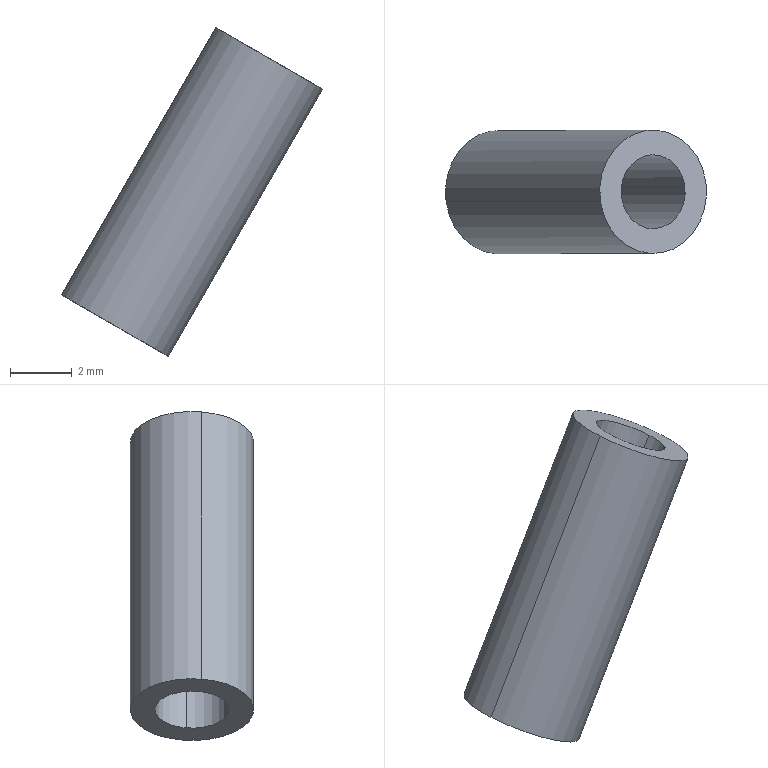Component | SolidWorks | WaterPipe5-1 | 1 solid | 6 faces | box 8.46 x 4 x 10.66 mm | volume 80 mm3 | cylinder 4 | plane 2 | commonest cylinder face diameters 2.4 x2 4 x2
build123d program:
from build123d import *

# Parameters (mm, degrees)
SCAN_THIN_FEATURE1_PROFILE_R   = 2
SCAN_THIN_FEATURE1_PROFILE_R_2 = 1.2


with BuildPart() as part:
    # Scan-Thin Feature1: sweep along a path in Sketch1
    with BuildLine(Plane.XY) as scan_thin_feature1_path:
        Line((0, 0), (10, 0))
    # Scan-Thin Feature1 profile (on start of the path) → Scan-Thin Feature1 (sweep)
    with BuildSketch(Plane(origin=(0, 0, 0), x_dir=(0, 0, 1), z_dir=(1, 0, 0))):
        Circle(SCAN_THIN_FEATURE1_PROFILE_R)
        Circle(SCAN_THIN_FEATURE1_PROFILE_R_2, mode=Mode.SUBTRACT)
    sweep(path=scan_thin_feature1_path.line)


solid = part.part

# Placed as in the assembly
solid = solid.moved(Location((35.951, 33.561, 104.495), (-176.489, 59.953, -3.04)))
STEP:
#1=CARTESIAN_POINT('',(1.375,1.314,4.137));
#2=VERTEX_POINT('',#1);
#3=CARTESIAN_POINT('',(1.456,1.329,4.091));
#4=VERTEX_POINT('',#3);
#5=CARTESIAN_POINT('',(1.415,1.321,4.114));
#6=DIRECTION('',(0.5,0.,0.866));
#7=DIRECTION('',(0.8553,0.1566,-0.4938));
#8=AXIS2_PLACEMENT_3D('',#5,#6,#7);
#9=CIRCLE('',#8,0.04724);
#10=EDGE_CURVE('',#2,#4,#9,.T.);
#11=ORIENTED_EDGE('',*,*,#10,.F.);
#12=CARTESIAN_POINT('',(1.572,1.314,4.478));
#13=VERTEX_POINT('',#12);
#14=CARTESIAN_POINT('',(1.375,1.314,4.137));
#15=DIRECTION('',(0.5,0.,0.866));
#16=VECTOR('',#15,39.37);
#17=LINE('',#14,#16);
#18=EDGE_CURVE('',#2,#13,#17,.T.);
#19=ORIENTED_EDGE('',*,*,#18,.T.);
#20=CARTESIAN_POINT('',(1.653,1.329,4.432));
#21=VERTEX_POINT('',#20);
#22=CARTESIAN_POINT('',(1.612,1.321,4.455));
#23=DIRECTION('',(0.5,0.,0.866));
#24=DIRECTION('',(0.8553,0.1566,-0.4938));
#25=AXIS2_PLACEMENT_3D('',#22,#23,#24);
#26=CIRCLE('',#25,0.04724);
#27=EDGE_CURVE('',#13,#21,#26,.T.);
#28=ORIENTED_EDGE('',*,*,#27,.T.);
#29=CARTESIAN_POINT('',(1.456,1.329,4.091));
#30=DIRECTION('',(0.5,0.,0.866));
#31=VECTOR('',#30,39.37);
#32=LINE('',#29,#31);
#33=EDGE_CURVE('',#4,#21,#32,.T.);
#34=ORIENTED_EDGE('',*,*,#33,.F.);
#35=EDGE_LOOP('',(#11,#19,#28,#34));
#36=FACE_OUTER_BOUND('',#35,.T.);
#37=CARTESIAN_POINT('',(1.415,1.321,4.114));
#38=DIRECTION('',(0.5,0.,0.866));
#39=DIRECTION('',(0.8553,0.1566,-0.4938));
#40=AXIS2_PLACEMENT_3D('',#37,#38,#39);
#41=CYLINDRICAL_SURFACE('',#40,0.04724);
#42=ADVANCED_FACE('',(#36),#41,.F.);
#43=CARTESIAN_POINT('',(1.483,1.334,4.075));
#44=VERTEX_POINT('',#43);
#45=CARTESIAN_POINT('',(1.348,1.309,4.153));
#46=VERTEX_POINT('',#45);
#47=CARTESIAN_POINT('',(1.415,1.321,4.114));
#48=DIRECTION('',(0.5,0.,0.866));
#49=DIRECTION('',(0.8553,0.1566,-0.4938));
#50=AXIS2_PLACEMENT_3D('',#47,#48,#49);
#51=CIRCLE('',#50,0.07874);
#52=EDGE_CURVE('',#44,#46,#51,.T.);
#53=ORIENTED_EDGE('',*,*,#52,.T.);
#54=CARTESIAN_POINT('',(1.545,1.309,4.494));
#55=VERTEX_POINT('',#54);
#56=CARTESIAN_POINT('',(1.348,1.309,4.153));
#57=DIRECTION('',(0.5,0.,0.866));
#58=VECTOR('',#57,39.37);
#59=LINE('',#56,#58);
#60=EDGE_CURVE('',#46,#55,#59,.T.);
#61=ORIENTED_EDGE('',*,*,#60,.T.);
#62=CARTESIAN_POINT('',(1.68,1.334,4.416));
#63=VERTEX_POINT('',#62);
#64=CARTESIAN_POINT('',(1.612,1.321,4.455));
#65=DIRECTION('',(0.5,0.,0.866));
#66=DIRECTION('',(0.8553,0.1566,-0.4938));
#67=AXIS2_PLACEMENT_3D('',#64,#65,#66);
#68=CIRCLE('',#67,0.07874);
#69=EDGE_CURVE('',#63,#55,#68,.T.);
#70=ORIENTED_EDGE('',*,*,#69,.F.);
#71=CARTESIAN_POINT('',(1.483,1.334,4.075));
#72=DIRECTION('',(0.5,0.,0.866));
#73=VECTOR('',#72,39.37);
#74=LINE('',#71,#73);
#75=EDGE_CURVE('',#44,#63,#74,.T.);
#76=ORIENTED_EDGE('',*,*,#75,.F.);
#77=EDGE_LOOP('',(#53,#61,#70,#76));
#78=FACE_OUTER_BOUND('',#77,.T.);
#79=CARTESIAN_POINT('',(1.415,1.321,4.114));
#80=DIRECTION('',(0.5,0.,0.866));
#81=DIRECTION('',(0.8553,0.1566,-0.4938));
#82=AXIS2_PLACEMENT_3D('',#79,#80,#81);
#83=CYLINDRICAL_SURFACE('',#82,0.07874);
#84=ADVANCED_FACE('',(#78),#83,.T.);
#85=ORIENTED_EDGE('',*,*,#60,.F.);
#86=CARTESIAN_POINT('',(1.415,1.321,4.114));
#87=DIRECTION('',(0.5,0.,0.866));
#88=DIRECTION('',(0.8553,0.1566,-0.4938));
#89=AXIS2_PLACEMENT_3D('',#86,#87,#88);
#90=CIRCLE('',#89,0.07874);
#91=EDGE_CURVE('',#46,#44,#90,.T.);
#92=ORIENTED_EDGE('',*,*,#91,.T.);
#93=ORIENTED_EDGE('',*,*,#75,.T.);
#94=CARTESIAN_POINT('',(1.612,1.321,4.455));
#95=DIRECTION('',(0.5,0.,0.866));
#96=DIRECTION('',(0.8553,0.1566,-0.4938));
#97=AXIS2_PLACEMENT_3D('',#94,#95,#96);
#98=CIRCLE('',#97,0.07874);
#99=EDGE_CURVE('',#55,#63,#98,.T.);
#100=ORIENTED_EDGE('',*,*,#99,.F.);
#101=EDGE_LOOP('',(#85,#92,#93,#100));
#102=FACE_OUTER_BOUND('',#101,.T.);
#103=CARTESIAN_POINT('',(1.415,1.321,4.114));
#104=DIRECTION('',(0.5,0.,0.866));
#105=DIRECTION('',(0.8553,0.1566,-0.4938));
#106=AXIS2_PLACEMENT_3D('',#103,#104,#105);
#107=CYLINDRICAL_SURFACE('',#106,0.07874);
#108=ADVANCED_FACE('',(#102),#107,.T.);
#109=CARTESIAN_POINT('',(1.612,1.321,4.455));
#110=DIRECTION('',(0.5,0.,0.866));
#111=DIRECTION('',(0.8553,0.1566,-0.4938));
#112=AXIS2_PLACEMENT_3D('',#109,#110,#111);
#113=CIRCLE('',#112,0.04724);
#114=EDGE_CURVE('',#21,#13,#113,.T.);
#115=ORIENTED_EDGE('',*,*,#114,.F.);
#116=ORIENTED_EDGE('',*,*,#27,.F.);
#117=EDGE_LOOP('',(#115,#116));
#118=FACE_BOUND('',#117,.T.);
#119=ORIENTED_EDGE('',*,*,#69,.T.);
#120=ORIENTED_EDGE('',*,*,#99,.T.);
#121=EDGE_LOOP('',(#119,#120));
#122=FACE_OUTER_BOUND('',#121,.T.);
#123=CARTESIAN_POINT('',(1.612,1.321,4.455));
#124=DIRECTION('',(0.5,0.,0.866));
#125=DIRECTION('',(0.8553,0.1566,-0.4938));
#126=AXIS2_PLACEMENT_3D('',#123,#124,#125);
#127=PLANE('',#126);
#128=ADVANCED_FACE('',(#118,#122),#127,.T.);
#129=CARTESIAN_POINT('',(1.415,1.321,4.114));
#130=DIRECTION('',(0.5,0.,0.866));
#131=DIRECTION('',(0.8553,0.1566,-0.4938));
#132=AXIS2_PLACEMENT_3D('',#129,#130,#131);
#133=CIRCLE('',#132,0.04724);
#134=EDGE_CURVE('',#4,#2,#133,.T.);
#135=ORIENTED_EDGE('',*,*,#134,.T.);
#136=ORIENTED_EDGE('',*,*,#10,.T.);
#137=EDGE_LOOP('',(#135,#136));
#138=FACE_BOUND('',#137,.T.);
#139=ORIENTED_EDGE('',*,*,#52,.F.);
#140=ORIENTED_EDGE('',*,*,#91,.F.);
#141=EDGE_LOOP('',(#139,#140));
#142=FACE_OUTER_BOUND('',#141,.T.);
#143=CARTESIAN_POINT('',(1.415,1.321,4.114));
#144=DIRECTION('',(0.5,0.,0.866));
#145=DIRECTION('',(0.8553,0.1566,-0.4938));
#146=AXIS2_PLACEMENT_3D('',#143,#144,#145);
#147=PLANE('',#146);
#148=ADVANCED_FACE('',(#138,#142),#147,.F.);
#149=ORIENTED_EDGE('',*,*,#18,.F.);
#150=ORIENTED_EDGE('',*,*,#134,.F.);
#151=ORIENTED_EDGE('',*,*,#33,.T.);
#152=ORIENTED_EDGE('',*,*,#114,.T.);
#153=EDGE_LOOP('',(#149,#150,#151,#152));
#154=FACE_OUTER_BOUND('',#153,.T.);
#155=CARTESIAN_POINT('',(1.415,1.321,4.114));
#156=DIRECTION('',(0.5,0.,0.866));
#157=DIRECTION('',(0.8553,0.1566,-0.4938));
#158=AXIS2_PLACEMENT_3D('',#155,#156,#157);
#159=CYLINDRICAL_SURFACE('',#158,0.04724);
#160=ADVANCED_FACE('',(#154),#159,.F.);
#161=CLOSED_SHELL('',(#42,#84,#108,#128,#148,#160));
#162=MANIFOLD_SOLID_BREP('',#161);
#163=CARTESIAN_POINT('',(0.,0.,0.));
#164=DIRECTION('',(0.,0.,1.));
#165=DIRECTION('',(1.,0.,0.));
#166=AXIS2_PLACEMENT_3D('',#163,#164,#165);
#167=(LENGTH_UNIT()NAMED_UNIT(*)SI_UNIT($,.METRE.));
#168=LENGTH_MEASURE_WITH_UNIT(LENGTH_MEASURE(0.0254),#167);
#169=DIMENSIONAL_EXPONENTS(1.,0.,0.,0.,0.,0.,0.);
#170=(CONVERSION_BASED_UNIT('',#168)LENGTH_UNIT()NAMED_UNIT(#169));
#171=UNCERTAINTY_MEASURE_WITH_UNIT(LENGTH_MEASURE(0.00001),#170,'','');
#172=(NAMED_UNIT(*)PLANE_ANGLE_UNIT()SI_UNIT($,.RADIAN.));
#173=(NAMED_UNIT(*)SI_UNIT($,.STERADIAN.)SOLID_ANGLE_UNIT());
#174=(GEOMETRIC_REPRESENTATION_CONTEXT(3)GLOBAL_UNCERTAINTY_ASSIGNED_CONTEXT((#171))GLOBAL_UNIT_ASSIGNED_CONTEXT((#170,#172,#173))REPRESENTATION_CONTEXT('',''));
#175=ADVANCED_BREP_SHAPE_REPRESENTATION('',(#162,#166),#174);
#176=COLOUR_RGB('',0.7922,0.8196,0.9333);
#177=FILL_AREA_STYLE_COLOUR('',#176);
#178=FILL_AREA_STYLE('',(#177));
#179=SURFACE_STYLE_FILL_AREA(#178);
#180=SURFACE_SIDE_STYLE('',(#179));
#181=SURFACE_STYLE_USAGE(.BOTH.,#180);
#182=PRESENTATION_STYLE_ASSIGNMENT((#181));
#183=STYLED_ITEM('',(#182),#162);
#184=PRESENTATION_LAYER_ASSIGNMENT('','',(#183));
#185=(LENGTH_UNIT()NAMED_UNIT(*)SI_UNIT($,.METRE.));
#186=LENGTH_MEASURE_WITH_UNIT(LENGTH_MEASURE(0.0254),#185);
#187=DIMENSIONAL_EXPONENTS(1.,0.,0.,0.,0.,0.,0.);
#188=(CONVERSION_BASED_UNIT('',#186)LENGTH_UNIT()NAMED_UNIT(#187));
#189=UNCERTAINTY_MEASURE_WITH_UNIT(LENGTH_MEASURE(0.00001),#188,'','');
#190=(NAMED_UNIT(*)PLANE_ANGLE_UNIT()SI_UNIT($,.RADIAN.));
#191=(NAMED_UNIT(*)SI_UNIT($,.STERADIAN.)SOLID_ANGLE_UNIT());
#192=(GEOMETRIC_REPRESENTATION_CONTEXT(3)GLOBAL_UNCERTAINTY_ASSIGNED_CONTEXT((#189))GLOBAL_UNIT_ASSIGNED_CONTEXT((#188,#190,#191))REPRESENTATION_CONTEXT('',''));
#193=MECHANICAL_DESIGN_GEOMETRIC_PRESENTATION_REPRESENTATION('',(#183),#192);